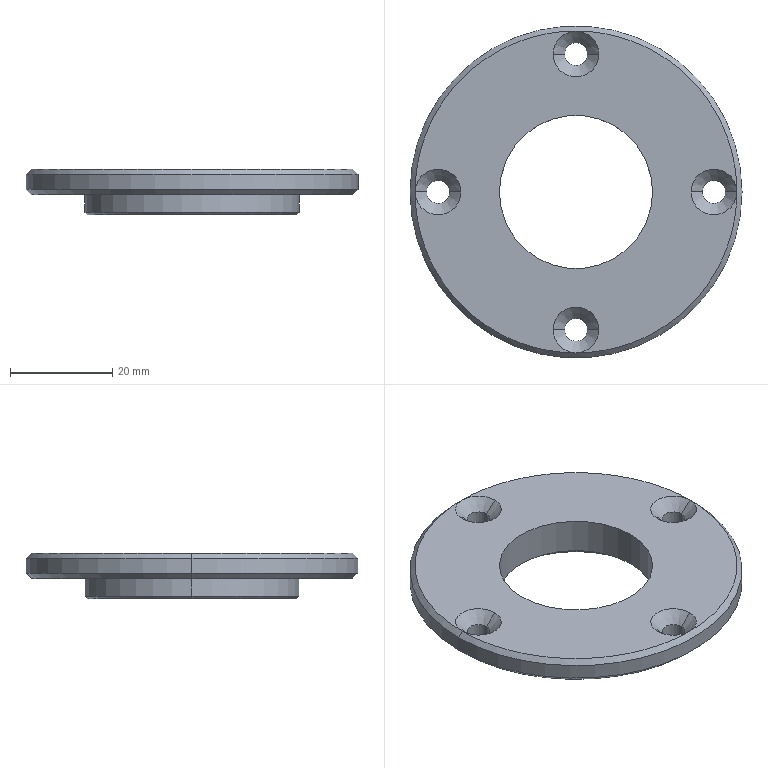Component | SolidWorks | TractionDriveWheelBearingEndCap-1 | 1 solid | 36 faces | box 65 x 65 x 9 mm | volume 14632 mm3 | cylinder 16 | cone 16 | plane 4 | commonest cylinder face diameters 4.5 x8 30 x2 34 x2 42 x2 65 x2
build123d program:
from build123d import *

# Parameters (mm, degrees)
CHAMFER1_SIZE                                        = 1
CHAMFER2_SIZE                                        = 0.5
M4_HEXAGON_SOCKET_COUNTERSUNK_HEAD_SCREW_D           = 4.5
M4_HEXAGON_SOCKET_COUNTERSUNK_HEAD_SCREW_CSINK_D     = 8.96
M4_HEXAGON_SOCKET_COUNTERSUNK_HEAD_SCREW_CSINK_ANGLE = 90
CIRPATTERN1_COUNT                                    = 4
SKETCH5_R                                            = 15
CUT_EXTRUDE1_DEPTH                                   = 47.835


with BuildPart() as part:
    # Sketch1 → Revolve1 (revolve)
    with BuildSketch(Plane(origin=(0, 0, 0), x_dir=(0, 0, -1), z_dir=(1, 0, 0)), mode=Mode.PRIVATE) as revolve1_sk:
        Polygon((0, 0), (0, 32.5), (5, 32.5), (5, 21), (9, 21), (9, 17), (7, 17), (7, 0), align=None)
    revolve(revolve1_sk.sketch.rotate(Axis((0, 0, 414.053), (0, 0, -1)), 90), axis=Axis((0, 0, 414.053), (0, 0, -1)))

    # Chamfer1
    chamfer1_edges = [part.edges().sort_by_distance(p)[0] for p in [
        (-32.5, 0, -5),
        (-32.5, 0, 0),
    ]]
    chamfer(chamfer1_edges, length=CHAMFER1_SIZE)

    # Chamfer2
    chamfer2_edges = [part.edges().sort_by_distance(p)[0] for p in [
        (-17, 0, -9),
        (-21, 0, -9),
    ]]
    chamfer(chamfer2_edges, length=CHAMFER2_SIZE)

    # M4 Hexagon Socket Countersunk Head Screw (through all)
    with Locations(Plane.XY):
        with Locations((0, 27)):
            m4_hexagon_socket_countersunk_head_screw = CounterSinkHole(M4_HEXAGON_SOCKET_COUNTERSUNK_HEAD_SCREW_D / 2, M4_HEXAGON_SOCKET_COUNTERSUNK_HEAD_SCREW_CSINK_D / 2, counter_sink_angle=M4_HEXAGON_SOCKET_COUNTERSUNK_HEAD_SCREW_CSINK_ANGLE)

    # CirPattern1: M4 Hexagon Socket Countersunk Head Screw ×4 about axis
    cirpattern1_axis = Axis((0, 0, 0), (0, 0, 1))
    for i in range(1, CIRPATTERN1_COUNT):
        add(m4_hexagon_socket_countersunk_head_screw.rotate(cirpattern1_axis, i * 360 / CIRPATTERN1_COUNT), mode=Mode.SUBTRACT)

    # Sketch5 → Cut-Extrude1 (cut, through all)
    with BuildSketch(Plane.XY):
        Circle(SKETCH5_R)
    extrude(amount=-CUT_EXTRUDE1_DEPTH, mode=Mode.SUBTRACT)


solid = part.part

# Placed as in the assembly
solid = solid.moved(Location((-299.507, -39.911, 646), (0, 0, 0)))
STEP:
#1=COLOUR_RGB('',0.7922,0.8196,0.9333);
#2=FILL_AREA_STYLE_COLOUR('',#1);
#3=FILL_AREA_STYLE('',(#2));
#4=SURFACE_STYLE_FILL_AREA(#3);
#5=SURFACE_SIDE_STYLE('',(#4));
#6=SURFACE_STYLE_USAGE(.BOTH.,#5);
#7=PRESENTATION_STYLE_ASSIGNMENT((#6));
#8=CARTESIAN_POINT('',(-12.382,-1.571,25.157));
#9=VERTEX_POINT('',#8);
#10=CARTESIAN_POINT('',(-11.201,-1.571,25.157));
#11=VERTEX_POINT('',#10);
#12=CARTESIAN_POINT('',(-11.792,-1.571,25.157));
#13=DIRECTION('',(0.,0.,1.));
#14=DIRECTION('',(1.,0.,0.));
#15=AXIS2_PLACEMENT_3D('',#12,#13,#14);
#16=CIRCLE('',#15,0.5906);
#17=EDGE_CURVE('',#9,#11,#16,.T.);
#18=ORIENTED_EDGE('',*,*,#17,.F.);
#19=CARTESIAN_POINT('',(-12.382,-1.571,25.433));
#20=VERTEX_POINT('',#19);
#21=CARTESIAN_POINT('',(-12.382,-1.571,25.079));
#22=DIRECTION('',(0.,0.,1.));
#23=VECTOR('',#22,39.37);
#24=LINE('',#21,#23);
#25=EDGE_CURVE('',#9,#20,#24,.T.);
#26=ORIENTED_EDGE('',*,*,#25,.T.);
#27=CARTESIAN_POINT('',(-11.201,-1.571,25.433));
#28=VERTEX_POINT('',#27);
#29=CARTESIAN_POINT('',(-11.792,-1.571,25.433));
#30=DIRECTION('',(0.,0.,1.));
#31=DIRECTION('',(1.,0.,0.));
#32=AXIS2_PLACEMENT_3D('',#29,#30,#31);
#33=CIRCLE('',#32,0.5906);
#34=EDGE_CURVE('',#20,#28,#33,.T.);
#35=ORIENTED_EDGE('',*,*,#34,.T.);
#36=CARTESIAN_POINT('',(-11.201,-1.571,25.079));
#37=DIRECTION('',(0.,0.,1.));
#38=VECTOR('',#37,39.37);
#39=LINE('',#36,#38);
#40=EDGE_CURVE('',#11,#28,#39,.T.);
#41=ORIENTED_EDGE('',*,*,#40,.F.);
#42=EDGE_LOOP('',(#18,#26,#35,#41));
#43=FACE_OUTER_BOUND('',#42,.T.);
#44=CARTESIAN_POINT('',(-11.792,-1.571,25.079));
#45=DIRECTION('',(0.,0.,1.));
#46=DIRECTION('',(1.,0.,0.));
#47=AXIS2_PLACEMENT_3D('',#44,#45,#46);
#48=CYLINDRICAL_SURFACE('',#47,0.5906);
#49=ADVANCED_FACE('',(#43),#48,.F.);
#50=CARTESIAN_POINT('',(-10.817,-1.571,25.345));
#51=VERTEX_POINT('',#50);
#52=CARTESIAN_POINT('',(-10.64,-1.571,25.345));
#53=VERTEX_POINT('',#52);
#54=CARTESIAN_POINT('',(-10.729,-1.571,25.345));
#55=DIRECTION('',(0.,0.,1.));
#56=DIRECTION('',(1.,0.,0.));
#57=AXIS2_PLACEMENT_3D('',#54,#55,#56);
#58=CIRCLE('',#57,0.08858);
#59=EDGE_CURVE('',#51,#53,#58,.T.);
#60=ORIENTED_EDGE('',*,*,#59,.F.);
#61=CARTESIAN_POINT('',(-10.905,-1.571,25.433));
#62=VERTEX_POINT('',#61);
#63=CARTESIAN_POINT('',(-10.905,-1.571,25.433));
#64=DIRECTION('',(-0.7071,0.,0.7071));
#65=VECTOR('',#64,39.37);
#66=LINE('',#63,#65);
#67=EDGE_CURVE('',#51,#62,#66,.T.);
#68=ORIENTED_EDGE('',*,*,#67,.T.);
#69=CARTESIAN_POINT('',(-10.552,-1.571,25.433));
#70=VERTEX_POINT('',#69);
#71=CARTESIAN_POINT('',(-10.729,-1.571,25.433));
#72=DIRECTION('',(0.,0.,1.));
#73=DIRECTION('',(1.,0.,0.));
#74=AXIS2_PLACEMENT_3D('',#71,#72,#73);
#75=CIRCLE('',#74,0.1764);
#76=EDGE_CURVE('',#62,#70,#75,.T.);
#77=ORIENTED_EDGE('',*,*,#76,.T.);
#78=CARTESIAN_POINT('',(-10.552,-1.571,25.433));
#79=DIRECTION('',(0.7071,0.,0.7071));
#80=VECTOR('',#79,39.37);
#81=LINE('',#78,#80);
#82=EDGE_CURVE('',#53,#70,#81,.T.);
#83=ORIENTED_EDGE('',*,*,#82,.F.);
#84=EDGE_LOOP('',(#60,#68,#77,#83));
#85=FACE_OUTER_BOUND('',#84,.T.);
#86=CARTESIAN_POINT('',(-10.729,-1.571,25.433));
#87=DIRECTION('',(0.,0.,1.));
#88=DIRECTION('',(1.,0.,0.));
#89=AXIS2_PLACEMENT_3D('',#86,#87,#88);
#90=CONICAL_SURFACE('',#89,0.1764,0.7854);
#91=ADVANCED_FACE('',(#85),#90,.F.);
#92=CARTESIAN_POINT('',(-10.817,-1.571,25.236));
#93=VERTEX_POINT('',#92);
#94=CARTESIAN_POINT('',(-10.64,-1.571,25.236));
#95=VERTEX_POINT('',#94);
#96=CARTESIAN_POINT('',(-10.729,-1.571,25.236));
#97=DIRECTION('',(0.,0.,1.));
#98=DIRECTION('',(1.,0.,0.));
#99=AXIS2_PLACEMENT_3D('',#96,#97,#98);
#100=CIRCLE('',#99,0.08858);
#101=EDGE_CURVE('',#93,#95,#100,.T.);
#102=ORIENTED_EDGE('',*,*,#101,.F.);
#103=CARTESIAN_POINT('',(-10.817,-1.571,25.433));
#104=DIRECTION('',(0.,0.,1.));
#105=VECTOR('',#104,39.37);
#106=LINE('',#103,#105);
#107=EDGE_CURVE('',#93,#51,#106,.T.);
#108=ORIENTED_EDGE('',*,*,#107,.T.);
#109=ORIENTED_EDGE('',*,*,#59,.T.);
#110=CARTESIAN_POINT('',(-10.64,-1.571,25.433));
#111=DIRECTION('',(0.,0.,1.));
#112=VECTOR('',#111,39.37);
#113=LINE('',#110,#112);
#114=EDGE_CURVE('',#95,#53,#113,.T.);
#115=ORIENTED_EDGE('',*,*,#114,.F.);
#116=EDGE_LOOP('',(#102,#108,#109,#115));
#117=FACE_OUTER_BOUND('',#116,.T.);
#118=CARTESIAN_POINT('',(-10.729,-1.571,25.433));
#119=DIRECTION('',(0.,0.,1.));
#120=DIRECTION('',(1.,0.,0.));
#121=AXIS2_PLACEMENT_3D('',#118,#119,#120);
#122=CYLINDRICAL_SURFACE('',#121,0.08858);
#123=ADVANCED_FACE('',(#117),#122,.F.);
#124=CARTESIAN_POINT('',(-11.88,-2.634,25.345));
#125=VERTEX_POINT('',#124);
#126=CARTESIAN_POINT('',(-11.703,-2.634,25.345));
#127=VERTEX_POINT('',#126);
#128=CARTESIAN_POINT('',(-11.792,-2.634,25.345));
#129=DIRECTION('',(0.,0.,1.));
#130=DIRECTION('',(1.,0.,0.));
#131=AXIS2_PLACEMENT_3D('',#128,#129,#130);
#132=CIRCLE('',#131,0.08858);
#133=EDGE_CURVE('',#125,#127,#132,.T.);
#134=ORIENTED_EDGE('',*,*,#133,.F.);
#135=CARTESIAN_POINT('',(-11.968,-2.634,25.433));
#136=VERTEX_POINT('',#135);
#137=CARTESIAN_POINT('',(-11.968,-2.634,25.433));
#138=DIRECTION('',(-0.7071,0.,0.7071));
#139=VECTOR('',#138,39.37);
#140=LINE('',#137,#139);
#141=EDGE_CURVE('',#125,#136,#140,.T.);
#142=ORIENTED_EDGE('',*,*,#141,.T.);
#143=CARTESIAN_POINT('',(-11.615,-2.634,25.433));
#144=VERTEX_POINT('',#143);
#145=CARTESIAN_POINT('',(-11.792,-2.634,25.433));
#146=DIRECTION('',(0.,0.,1.));
#147=DIRECTION('',(1.,0.,0.));
#148=AXIS2_PLACEMENT_3D('',#145,#146,#147);
#149=CIRCLE('',#148,0.1764);
#150=EDGE_CURVE('',#136,#144,#149,.T.);
#151=ORIENTED_EDGE('',*,*,#150,.T.);
#152=CARTESIAN_POINT('',(-11.615,-2.634,25.433));
#153=DIRECTION('',(0.7071,0.,0.7071));
#154=VECTOR('',#153,39.37);
#155=LINE('',#152,#154);
#156=EDGE_CURVE('',#127,#144,#155,.T.);
#157=ORIENTED_EDGE('',*,*,#156,.F.);
#158=EDGE_LOOP('',(#134,#142,#151,#157));
#159=FACE_OUTER_BOUND('',#158,.T.);
#160=CARTESIAN_POINT('',(-11.792,-2.634,25.433));
#161=DIRECTION('',(0.,0.,1.));
#162=DIRECTION('',(1.,0.,0.));
#163=AXIS2_PLACEMENT_3D('',#160,#161,#162);
#164=CONICAL_SURFACE('',#163,0.1764,0.7854);
#165=ADVANCED_FACE('',(#159),#164,.F.);
#166=CARTESIAN_POINT('',(-11.88,-2.634,25.236));
#167=VERTEX_POINT('',#166);
#168=CARTESIAN_POINT('',(-11.703,-2.634,25.236));
#169=VERTEX_POINT('',#168);
#170=CARTESIAN_POINT('',(-11.792,-2.634,25.236));
#171=DIRECTION('',(0.,0.,1.));
#172=DIRECTION('',(1.,0.,0.));
#173=AXIS2_PLACEMENT_3D('',#170,#171,#172);
#174=CIRCLE('',#173,0.08858);
#175=EDGE_CURVE('',#167,#169,#174,.T.);
#176=ORIENTED_EDGE('',*,*,#175,.F.);
#177=CARTESIAN_POINT('',(-11.88,-2.634,25.433));
#178=DIRECTION('',(0.,0.,1.));
#179=VECTOR('',#178,39.37);
#180=LINE('',#177,#179);
#181=EDGE_CURVE('',#167,#125,#180,.T.);
#182=ORIENTED_EDGE('',*,*,#181,.T.);
#183=ORIENTED_EDGE('',*,*,#133,.T.);
#184=CARTESIAN_POINT('',(-11.703,-2.634,25.433));
#185=DIRECTION('',(0.,0.,1.));
#186=VECTOR('',#185,39.37);
#187=LINE('',#184,#186);
#188=EDGE_CURVE('',#169,#127,#187,.T.);
#189=ORIENTED_EDGE('',*,*,#188,.F.);
#190=EDGE_LOOP('',(#176,#182,#183,#189));
#191=FACE_OUTER_BOUND('',#190,.T.);
#192=CARTESIAN_POINT('',(-11.792,-2.634,25.433));
#193=DIRECTION('',(0.,0.,1.));
#194=DIRECTION('',(1.,0.,0.));
#195=AXIS2_PLACEMENT_3D('',#192,#193,#194);
#196=CYLINDRICAL_SURFACE('',#195,0.08858);
#197=ADVANCED_FACE('',(#191),#196,.F.);
#198=CARTESIAN_POINT('',(-12.943,-1.571,25.345));
#199=VERTEX_POINT('',#198);
#200=CARTESIAN_POINT('',(-12.766,-1.571,25.345));
#201=VERTEX_POINT('',#200);
#202=CARTESIAN_POINT('',(-12.855,-1.571,25.345));
#203=DIRECTION('',(0.,0.,1.));
#204=DIRECTION('',(1.,0.,0.));
#205=AXIS2_PLACEMENT_3D('',#202,#203,#204);
#206=CIRCLE('',#205,0.08858);
#207=EDGE_CURVE('',#199,#201,#206,.T.);
#208=ORIENTED_EDGE('',*,*,#207,.F.);
#209=CARTESIAN_POINT('',(-13.031,-1.571,25.433));
#210=VERTEX_POINT('',#209);
#211=CARTESIAN_POINT('',(-13.031,-1.571,25.433));
#212=DIRECTION('',(-0.7071,0.,0.7071));
#213=VECTOR('',#212,39.37);
#214=LINE('',#211,#213);
#215=EDGE_CURVE('',#199,#210,#214,.T.);
#216=ORIENTED_EDGE('',*,*,#215,.T.);
#217=CARTESIAN_POINT('',(-12.678,-1.571,25.433));
#218=VERTEX_POINT('',#217);
#219=CARTESIAN_POINT('',(-12.855,-1.571,25.433));
#220=DIRECTION('',(0.,0.,1.));
#221=DIRECTION('',(1.,0.,0.));
#222=AXIS2_PLACEMENT_3D('',#219,#220,#221);
#223=CIRCLE('',#222,0.1764);
#224=EDGE_CURVE('',#210,#218,#223,.T.);
#225=ORIENTED_EDGE('',*,*,#224,.T.);
#226=CARTESIAN_POINT('',(-12.678,-1.571,25.433));
#227=DIRECTION('',(0.7071,0.,0.7071));
#228=VECTOR('',#227,39.37);
#229=LINE('',#226,#228);
#230=EDGE_CURVE('',#201,#218,#229,.T.);
#231=ORIENTED_EDGE('',*,*,#230,.F.);
#232=EDGE_LOOP('',(#208,#216,#225,#231));
#233=FACE_OUTER_BOUND('',#232,.T.);
#234=CARTESIAN_POINT('',(-12.855,-1.571,25.433));
#235=DIRECTION('',(0.,0.,1.));
#236=DIRECTION('',(1.,0.,0.));
#237=AXIS2_PLACEMENT_3D('',#234,#235,#236);
#238=CONICAL_SURFACE('',#237,0.1764,0.7854);
#239=ADVANCED_FACE('',(#233),#238,.F.);
#240=CARTESIAN_POINT('',(-12.943,-1.571,25.236));
#241=VERTEX_POINT('',#240);
#242=CARTESIAN_POINT('',(-12.766,-1.571,25.236));
#243=VERTEX_POINT('',#242);
#244=CARTESIAN_POINT('',(-12.855,-1.571,25.236));
#245=DIRECTION('',(0.,0.,1.));
#246=DIRECTION('',(1.,0.,0.));
#247=AXIS2_PLACEMENT_3D('',#244,#245,#246);
#248=CIRCLE('',#247,0.08858);
#249=EDGE_CURVE('',#241,#243,#248,.T.);
#250=ORIENTED_EDGE('',*,*,#249,.F.);
#251=CARTESIAN_POINT('',(-12.943,-1.571,25.433));
#252=DIRECTION('',(0.,0.,1.));
#253=VECTOR('',#252,39.37);
#254=LINE('',#251,#253);
#255=EDGE_CURVE('',#241,#199,#254,.T.);
#256=ORIENTED_EDGE('',*,*,#255,.T.);
#257=ORIENTED_EDGE('',*,*,#207,.T.);
#258=CARTESIAN_POINT('',(-12.766,-1.571,25.433));
#259=DIRECTION('',(0.,0.,1.));
#260=VECTOR('',#259,39.37);
#261=LINE('',#258,#260);
#262=EDGE_CURVE('',#243,#201,#261,.T.);
#263=ORIENTED_EDGE('',*,*,#262,.F.);
#264=EDGE_LOOP('',(#250,#256,#257,#263));
#265=FACE_OUTER_BOUND('',#264,.T.);
#266=CARTESIAN_POINT('',(-12.855,-1.571,25.433));
#267=DIRECTION('',(0.,0.,1.));
#268=DIRECTION('',(1.,0.,0.));
#269=AXIS2_PLACEMENT_3D('',#266,#267,#268);
#270=CYLINDRICAL_SURFACE('',#269,0.08858);
#271=ADVANCED_FACE('',(#265),#270,.F.);
#272=CARTESIAN_POINT('',(-11.88,-0.5083,25.345));
#273=VERTEX_POINT('',#272);
#274=CARTESIAN_POINT('',(-11.703,-0.5083,25.345));
#275=VERTEX_POINT('',#274);
#276=CARTESIAN_POINT('',(-11.792,-0.5083,25.345));
#277=DIRECTION('',(0.,0.,1.));
#278=DIRECTION('',(1.,0.,0.));
#279=AXIS2_PLACEMENT_3D('',#276,#277,#278);
#280=CIRCLE('',#279,0.08858);
#281=EDGE_CURVE('',#273,#275,#280,.T.);
#282=ORIENTED_EDGE('',*,*,#281,.F.);
#283=CARTESIAN_POINT('',(-11.968,-0.5083,25.433));
#284=VERTEX_POINT('',#283);
#285=CARTESIAN_POINT('',(-11.968,-0.5083,25.433));
#286=DIRECTION('',(-0.7071,0.,0.7071));
#287=VECTOR('',#286,39.37);
#288=LINE('',#285,#287);
#289=EDGE_CURVE('',#273,#284,#288,.T.);
#290=ORIENTED_EDGE('',*,*,#289,.T.);
#291=CARTESIAN_POINT('',(-11.615,-0.5083,25.433));
#292=VERTEX_POINT('',#291);
#293=CARTESIAN_POINT('',(-11.792,-0.5083,25.433));
#294=DIRECTION('',(0.,0.,1.));
#295=DIRECTION('',(1.,0.,0.));
#296=AXIS2_PLACEMENT_3D('',#293,#294,#295);
#297=CIRCLE('',#296,0.1764);
#298=EDGE_CURVE('',#284,#292,#297,.T.);
#299=ORIENTED_EDGE('',*,*,#298,.T.);
#300=CARTESIAN_POINT('',(-11.615,-0.5083,25.433));
#301=DIRECTION('',(0.7071,0.,0.7071));
#302=VECTOR('',#301,39.37);
#303=LINE('',#300,#302);
#304=EDGE_CURVE('',#275,#292,#303,.T.);
#305=ORIENTED_EDGE('',*,*,#304,.F.);
#306=EDGE_LOOP('',(#282,#290,#299,#305));
#307=FACE_OUTER_BOUND('',#306,.T.);
#308=CARTESIAN_POINT('',(-11.792,-0.5083,25.433));
#309=DIRECTION('',(0.,0.,1.));
#310=DIRECTION('',(1.,0.,0.));
#311=AXIS2_PLACEMENT_3D('',#308,#309,#310);
#312=CONICAL_SURFACE('',#311,0.1764,0.7854);
#313=ADVANCED_FACE('',(#307),#312,.F.);
#314=CARTESIAN_POINT('',(-11.88,-0.5083,25.236));
#315=VERTEX_POINT('',#314);
#316=CARTESIAN_POINT('',(-11.703,-0.5083,25.236));
#317=VERTEX_POINT('',#316);
#318=CARTESIAN_POINT('',(-11.792,-0.5083,25.236));
#319=DIRECTION('',(0.,0.,1.));
#320=DIRECTION('',(1.,0.,0.));
#321=AXIS2_PLACEMENT_3D('',#318,#319,#320);
#322=CIRCLE('',#321,0.08858);
#323=EDGE_CURVE('',#315,#317,#322,.T.);
#324=ORIENTED_EDGE('',*,*,#323,.F.);
#325=CARTESIAN_POINT('',(-11.88,-0.5083,25.433));
#326=DIRECTION('',(0.,0.,1.));
#327=VECTOR('',#326,39.37);
#328=LINE('',#325,#327);
#329=EDGE_CURVE('',#315,#273,#328,.T.);
#330=ORIENTED_EDGE('',*,*,#329,.T.);
#331=ORIENTED_EDGE('',*,*,#281,.T.);
#332=CARTESIAN_POINT('',(-11.703,-0.5083,25.433));
#333=DIRECTION('',(0.,0.,1.));
#334=VECTOR('',#333,39.37);
#335=LINE('',#332,#334);
#336=EDGE_CURVE('',#317,#275,#335,.T.);
#337=ORIENTED_EDGE('',*,*,#336,.F.);
#338=EDGE_LOOP('',(#324,#330,#331,#337));
#339=FACE_OUTER_BOUND('',#338,.T.);
#340=CARTESIAN_POINT('',(-11.792,-0.5083,25.433));
#341=DIRECTION('',(0.,0.,1.));
#342=DIRECTION('',(1.,0.,0.));
#343=AXIS2_PLACEMENT_3D('',#340,#341,#342);
#344=CYLINDRICAL_SURFACE('',#343,0.08858);
#345=ADVANCED_FACE('',(#339),#344,.F.);
#346=CARTESIAN_POINT('',(-11.122,-1.571,25.098));
#347=VERTEX_POINT('',#346);
#348=CARTESIAN_POINT('',(-12.461,-1.571,25.098));
#349=VERTEX_POINT('',#348);
#350=CARTESIAN_POINT('',(-11.792,-1.571,25.098));
#351=DIRECTION('',(0.,0.,-1.));
#352=DIRECTION('',(1.,0.,0.));
#353=AXIS2_PLACEMENT_3D('',#350,#351,#352);
#354=CIRCLE('',#353,0.6693);
#355=EDGE_CURVE('',#347,#349,#354,.T.);
#356=ORIENTED_EDGE('',*,*,#355,.F.);
#357=CARTESIAN_POINT('',(-11.103,-1.571,25.079));
#358=VERTEX_POINT('',#357);
#359=CARTESIAN_POINT('',(-11.103,-1.571,25.079));
#360=DIRECTION('',(0.7071,0.,-0.7071));
#361=VECTOR('',#360,39.37);
#362=LINE('',#359,#361);
#363=EDGE_CURVE('',#347,#358,#362,.T.);
#364=ORIENTED_EDGE('',*,*,#363,.T.);
#365=CARTESIAN_POINT('',(-12.481,-1.571,25.079));
#366=VERTEX_POINT('',#365);
#367=CARTESIAN_POINT('',(-11.792,-1.571,25.079));
#368=DIRECTION('',(0.,0.,1.));
#369=DIRECTION('',(1.,0.,0.));
#370=AXIS2_PLACEMENT_3D('',#367,#368,#369);
#371=CIRCLE('',#370,0.689);
#372=EDGE_CURVE('',#366,#358,#371,.T.);
#373=ORIENTED_EDGE('',*,*,#372,.F.);
#374=CARTESIAN_POINT('',(-12.481,-1.571,25.079));
#375=DIRECTION('',(-0.7071,0.,-0.7071));
#376=VECTOR('',#375,39.37);
#377=LINE('',#374,#376);
#378=EDGE_CURVE('',#349,#366,#377,.T.);
#379=ORIENTED_EDGE('',*,*,#378,.F.);
#380=EDGE_LOOP('',(#356,#364,#373,#379));
#381=FACE_OUTER_BOUND('',#380,.T.);
#382=CARTESIAN_POINT('',(-11.792,-1.571,25.079));
#383=DIRECTION('',(0.,0.,-1.));
#384=DIRECTION('',(-1.,0.,0.));
#385=AXIS2_PLACEMENT_3D('',#382,#383,#384);
#386=CONICAL_SURFACE('',#385,0.689,0.7854);
#387=ADVANCED_FACE('',(#381),#386,.F.);
#388=CARTESIAN_POINT('',(-12.599,-1.571,25.079));
#389=VERTEX_POINT('',#388);
#390=CARTESIAN_POINT('',(-10.985,-1.571,25.079));
#391=VERTEX_POINT('',#390);
#392=CARTESIAN_POINT('',(-11.792,-1.571,25.079));
#393=DIRECTION('',(0.,0.,-1.));
#394=DIRECTION('',(1.,0.,0.));
#395=AXIS2_PLACEMENT_3D('',#392,#393,#394);
#396=CIRCLE('',#395,0.8071);
#397=EDGE_CURVE('',#389,#391,#396,.T.);
#398=ORIENTED_EDGE('',*,*,#397,.F.);
#399=CARTESIAN_POINT('',(-12.618,-1.571,25.098));
#400=VERTEX_POINT('',#399);
#401=CARTESIAN_POINT('',(-12.618,-1.571,25.098));
#402=DIRECTION('',(-0.7071,0.,0.7071));
#403=VECTOR('',#402,39.37);
#404=LINE('',#401,#403);
#405=EDGE_CURVE('',#389,#400,#404,.T.);
#406=ORIENTED_EDGE('',*,*,#405,.T.);
#407=CARTESIAN_POINT('',(-10.965,-1.571,25.098));
#408=VERTEX_POINT('',#407);
#409=CARTESIAN_POINT('',(-11.792,-1.571,25.098));
#410=DIRECTION('',(0.,0.,1.));
#411=DIRECTION('',(1.,0.,0.));
#412=AXIS2_PLACEMENT_3D('',#409,#410,#411);
#413=CIRCLE('',#412,0.8268);
#414=EDGE_CURVE('',#408,#400,#413,.T.);
#415=ORIENTED_EDGE('',*,*,#414,.F.);
#416=CARTESIAN_POINT('',(-10.965,-1.571,25.098));
#417=DIRECTION('',(0.7071,0.,0.7071));
#418=VECTOR('',#417,39.37);
#419=LINE('',#416,#418);
#420=EDGE_CURVE('',#391,#408,#419,.T.);
#421=ORIENTED_EDGE('',*,*,#420,.F.);
#422=EDGE_LOOP('',(#398,#406,#415,#421));
#423=FACE_OUTER_BOUND('',#422,.T.);
#424=CARTESIAN_POINT('',(-11.792,-1.571,25.098));
#425=DIRECTION('',(0.,0.,1.));
#426=DIRECTION('',(1.,0.,0.));
#427=AXIS2_PLACEMENT_3D('',#424,#425,#426);
#428=CONICAL_SURFACE('',#427,0.8268,0.7854);
#429=ADVANCED_FACE('',(#423),#428,.T.);
#430=CARTESIAN_POINT('',(-13.032,-1.571,25.236));
#431=VERTEX_POINT('',#430);
#432=CARTESIAN_POINT('',(-10.551,-1.571,25.236));
#433=VERTEX_POINT('',#432);
#434=CARTESIAN_POINT('',(-11.792,-1.571,25.236));
#435=DIRECTION('',(0.,0.,-1.));
#436=DIRECTION('',(1.,0.,0.));
#437=AXIS2_PLACEMENT_3D('',#434,#435,#436);
#438=CIRCLE('',#437,1.24);
#439=EDGE_CURVE('',#431,#433,#438,.T.);
#440=ORIENTED_EDGE('',*,*,#439,.F.);
#441=CARTESIAN_POINT('',(-13.071,-1.571,25.276));
#442=VERTEX_POINT('',#441);
#443=CARTESIAN_POINT('',(-13.071,-1.571,25.276));
#444=DIRECTION('',(-0.7071,0.,0.7071));
#445=VECTOR('',#444,39.37);
#446=LINE('',#443,#445);
#447=EDGE_CURVE('',#431,#442,#446,.T.);
#448=ORIENTED_EDGE('',*,*,#447,.T.);
#449=CARTESIAN_POINT('',(-10.512,-1.571,25.276));
#450=VERTEX_POINT('',#449);
#451=CARTESIAN_POINT('',(-11.792,-1.571,25.276));
#452=DIRECTION('',(0.,0.,1.));
#453=DIRECTION('',(1.,0.,0.));
#454=AXIS2_PLACEMENT_3D('',#451,#452,#453);
#455=CIRCLE('',#454,1.28);
#456=EDGE_CURVE('',#450,#442,#455,.T.);
#457=ORIENTED_EDGE('',*,*,#456,.F.);
#458=CARTESIAN_POINT('',(-10.512,-1.571,25.276));
#459=DIRECTION('',(0.7071,0.,0.7071));
#460=VECTOR('',#459,39.37);
#461=LINE('',#458,#460);
#462=EDGE_CURVE('',#433,#450,#461,.T.);
#463=ORIENTED_EDGE('',*,*,#462,.F.);
#464=EDGE_LOOP('',(#440,#448,#457,#463));
#465=FACE_OUTER_BOUND('',#464,.T.);
#466=CARTESIAN_POINT('',(-11.792,-1.571,25.276));
#467=DIRECTION('',(0.,0.,1.));
#468=DIRECTION('',(1.,0.,0.));
#469=AXIS2_PLACEMENT_3D('',#466,#467,#468);
#470=CONICAL_SURFACE('',#469,1.28,0.7854);
#471=ADVANCED_FACE('',(#465),#470,.T.);
#472=CARTESIAN_POINT('',(-10.551,-1.571,25.433));
#473=VERTEX_POINT('',#472);
#474=CARTESIAN_POINT('',(-13.032,-1.571,25.433));
#475=VERTEX_POINT('',#474);
#476=CARTESIAN_POINT('',(-11.792,-1.571,25.433));
#477=DIRECTION('',(0.,0.,1.));
#478=DIRECTION('',(-1.,0.,0.));
#479=AXIS2_PLACEMENT_3D('',#476,#477,#478);
#480=CIRCLE('',#479,1.24);
#481=EDGE_CURVE('',#473,#475,#480,.T.);
#482=ORIENTED_EDGE('',*,*,#481,.F.);
#483=CARTESIAN_POINT('',(-10.512,-1.571,25.394));
#484=VERTEX_POINT('',#483);
#485=CARTESIAN_POINT('',(-10.551,-1.571,25.433));
#486=DIRECTION('',(0.7071,0.,-0.7071));
#487=VECTOR('',#486,39.37);
#488=LINE('',#485,#487);
#489=EDGE_CURVE('',#473,#484,#488,.T.);
#490=ORIENTED_EDGE('',*,*,#489,.T.);
#491=CARTESIAN_POINT('',(-13.071,-1.571,25.394));
#492=VERTEX_POINT('',#491);
#493=CARTESIAN_POINT('',(-11.792,-1.571,25.394));
#494=DIRECTION('',(0.,0.,-1.));
#495=DIRECTION('',(-1.,0.,0.));
#496=AXIS2_PLACEMENT_3D('',#493,#494,#495);
#497=CIRCLE('',#496,1.28);
#498=EDGE_CURVE('',#492,#484,#497,.T.);
#499=ORIENTED_EDGE('',*,*,#498,.F.);
#500=CARTESIAN_POINT('',(-13.032,-1.571,25.433));
#501=DIRECTION('',(-0.7071,0.,-0.7071));
#502=VECTOR('',#501,39.37);
#503=LINE('',#500,#502);
#504=EDGE_CURVE('',#475,#492,#503,.T.);
#505=ORIENTED_EDGE('',*,*,#504,.F.);
#506=EDGE_LOOP('',(#482,#490,#499,#505));
#507=FACE_OUTER_BOUND('',#506,.T.);
#508=CARTESIAN_POINT('',(-11.792,-1.571,25.433));
#509=DIRECTION('',(0.,0.,-1.));
#510=DIRECTION('',(-1.,0.,0.));
#511=AXIS2_PLACEMENT_3D('',#508,#509,#510);
#512=CONICAL_SURFACE('',#511,1.24,0.7854);
#513=ADVANCED_FACE('',(#507),#512,.T.);
#514=ORIENTED_EDGE('',*,*,#355,.T.);
#515=CARTESIAN_POINT('',(-12.461,-1.571,25.157));
#516=VERTEX_POINT('',#515);
#517=CARTESIAN_POINT('',(-12.461,-1.571,41.734));
#518=DIRECTION('',(0.,0.,1.));
#519=VECTOR('',#518,39.37);
#520=LINE('',#517,#519);
#521=EDGE_CURVE('',#349,#516,#520,.T.);
#522=ORIENTED_EDGE('',*,*,#521,.T.);
#523=CARTESIAN_POINT('',(-11.122,-1.571,25.157));
#524=VERTEX_POINT('',#523);
#525=CARTESIAN_POINT('',(-11.792,-1.571,25.157));
#526=DIRECTION('',(0.,0.,1.));
#527=DIRECTION('',(1.,0.,0.));
#528=AXIS2_PLACEMENT_3D('',#525,#526,#527);
#529=CIRCLE('',#528,0.6693);
#530=EDGE_CURVE('',#516,#524,#529,.T.);
#531=ORIENTED_EDGE('',*,*,#530,.T.);
#532=CARTESIAN_POINT('',(-11.122,-1.571,41.734));
#533=DIRECTION('',(0.,0.,1.));
#534=VECTOR('',#533,39.37);
#535=LINE('',#532,#534);
#536=EDGE_CURVE('',#347,#524,#535,.T.);
#537=ORIENTED_EDGE('',*,*,#536,.F.);
#538=EDGE_LOOP('',(#514,#522,#531,#537));
#539=FACE_OUTER_BOUND('',#538,.T.);
#540=CARTESIAN_POINT('',(-11.792,-1.571,41.734));
#541=DIRECTION('',(0.,0.,1.));
#542=DIRECTION('',(1.,0.,0.));
#543=AXIS2_PLACEMENT_3D('',#540,#541,#542);
#544=CYLINDRICAL_SURFACE('',#543,0.6693);
#545=ADVANCED_FACE('',(#539),#544,.F.);
#546=ORIENTED_EDGE('',*,*,#414,.T.);
#547=CARTESIAN_POINT('',(-12.618,-1.571,25.236));
#548=VERTEX_POINT('',#547);
#549=CARTESIAN_POINT('',(-12.618,-1.571,41.734));
#550=DIRECTION('',(0.,0.,1.));
#551=VECTOR('',#550,39.37);
#552=LINE('',#549,#551);
#553=EDGE_CURVE('',#400,#548,#552,.T.);
#554=ORIENTED_EDGE('',*,*,#553,.T.);
#555=CARTESIAN_POINT('',(-10.965,-1.571,25.236));
#556=VERTEX_POINT('',#555);
#557=CARTESIAN_POINT('',(-11.792,-1.571,25.236));
#558=DIRECTION('',(0.,0.,1.));
#559=DIRECTION('',(1.,0.,0.));
#560=AXIS2_PLACEMENT_3D('',#557,#558,#559);
#561=CIRCLE('',#560,0.8268);
#562=EDGE_CURVE('',#556,#548,#561,.T.);
#563=ORIENTED_EDGE('',*,*,#562,.F.);
#564=CARTESIAN_POINT('',(-10.965,-1.571,41.734));
#565=DIRECTION('',(0.,0.,1.));
#566=VECTOR('',#565,39.37);
#567=LINE('',#564,#566);
#568=EDGE_CURVE('',#408,#556,#567,.T.);
#569=ORIENTED_EDGE('',*,*,#568,.F.);
#570=EDGE_LOOP('',(#546,#554,#563,#569));
#571=FACE_OUTER_BOUND('',#570,.T.);
#572=CARTESIAN_POINT('',(-11.792,-1.571,41.734));
#573=DIRECTION('',(0.,0.,1.));
#574=DIRECTION('',(1.,0.,0.));
#575=AXIS2_PLACEMENT_3D('',#572,#573,#574);
#576=CYLINDRICAL_SURFACE('',#575,0.8268);
#577=ADVANCED_FACE('',(#571),#576,.T.);
#578=ORIENTED_EDGE('',*,*,#456,.T.);
#579=CARTESIAN_POINT('',(-13.071,-1.571,41.734));
#580=DIRECTION('',(0.,0.,1.));
#581=VECTOR('',#580,39.37);
#582=LINE('',#579,#581);
#583=EDGE_CURVE('',#442,#492,#582,.T.);
#584=ORIENTED_EDGE('',*,*,#583,.T.);
#585=ORIENTED_EDGE('',*,*,#498,.T.);
#586=CARTESIAN_POINT('',(-10.512,-1.571,41.734));
#587=DIRECTION('',(0.,0.,1.));
#588=VECTOR('',#587,39.37);
#589=LINE('',#586,#588);
#590=EDGE_CURVE('',#450,#484,#589,.T.);
#591=ORIENTED_EDGE('',*,*,#590,.F.);
#592=EDGE_LOOP('',(#578,#584,#585,#591));
#593=FACE_OUTER_BOUND('',#592,.T.);
#594=CARTESIAN_POINT('',(-11.792,-1.571,41.734));
#595=DIRECTION('',(0.,0.,1.));
#596=DIRECTION('',(1.,0.,0.));
#597=AXIS2_PLACEMENT_3D('',#594,#595,#596);
#598=CYLINDRICAL_SURFACE('',#597,1.28);
#599=ADVANCED_FACE('',(#593),#598,.T.);
#600=CARTESIAN_POINT('',(-11.792,-1.571,25.433));
#601=DIRECTION('',(0.,0.,1.));
#602=DIRECTION('',(1.,0.,0.));
#603=AXIS2_PLACEMENT_3D('',#600,#601,#602);
#604=CIRCLE('',#603,0.5906);
#605=EDGE_CURVE('',#28,#20,#604,.T.);
#606=ORIENTED_EDGE('',*,*,#605,.F.);
#607=ORIENTED_EDGE('',*,*,#34,.F.);
#608=EDGE_LOOP('',(#606,#607));
#609=FACE_BOUND('',#608,.T.);
#610=CARTESIAN_POINT('',(-10.729,-1.571,25.433));
#611=DIRECTION('',(0.,0.,1.));
#612=DIRECTION('',(1.,0.,0.));
#613=AXIS2_PLACEMENT_3D('',#610,#611,#612);
#614=CIRCLE('',#613,0.1764);
#615=EDGE_CURVE('',#70,#62,#614,.T.);
#616=ORIENTED_EDGE('',*,*,#615,.F.);
#617=ORIENTED_EDGE('',*,*,#76,.F.);
#618=EDGE_LOOP('',(#616,#617));
#619=FACE_BOUND('',#618,.T.);
#620=CARTESIAN_POINT('',(-11.792,-2.634,25.433));
#621=DIRECTION('',(0.,0.,1.));
#622=DIRECTION('',(1.,0.,0.));
#623=AXIS2_PLACEMENT_3D('',#620,#621,#622);
#624=CIRCLE('',#623,0.1764);
#625=EDGE_CURVE('',#144,#136,#624,.T.);
#626=ORIENTED_EDGE('',*,*,#625,.F.);
#627=ORIENTED_EDGE('',*,*,#150,.F.);
#628=EDGE_LOOP('',(#626,#627));
#629=FACE_BOUND('',#628,.T.);
#630=CARTESIAN_POINT('',(-12.855,-1.571,25.433));
#631=DIRECTION('',(0.,0.,1.));
#632=DIRECTION('',(1.,0.,0.));
#633=AXIS2_PLACEMENT_3D('',#630,#631,#632);
#634=CIRCLE('',#633,0.1764);
#635=EDGE_CURVE('',#218,#210,#634,.T.);
#636=ORIENTED_EDGE('',*,*,#635,.F.);
#637=ORIENTED_EDGE('',*,*,#224,.F.);
#638=EDGE_LOOP('',(#636,#637));
#639=FACE_BOUND('',#638,.T.);
#640=CARTESIAN_POINT('',(-11.792,-0.5083,25.433));
#641=DIRECTION('',(0.,0.,1.));
#642=DIRECTION('',(1.,0.,0.));
#643=AXIS2_PLACEMENT_3D('',#640,#641,#642);
#644=CIRCLE('',#643,0.1764);
#645=EDGE_CURVE('',#292,#284,#644,.T.);
#646=ORIENTED_EDGE('',*,*,#645,.F.);
#647=ORIENTED_EDGE('',*,*,#298,.F.);
#648=EDGE_LOOP('',(#646,#647));
#649=FACE_BOUND('',#648,.T.);
#650=CARTESIAN_POINT('',(-11.792,-1.571,25.433));
#651=DIRECTION('',(0.,0.,1.));
#652=DIRECTION('',(-1.,0.,0.));
#653=AXIS2_PLACEMENT_3D('',#650,#651,#652);
#654=CIRCLE('',#653,1.24);
#655=EDGE_CURVE('',#475,#473,#654,.T.);
#656=ORIENTED_EDGE('',*,*,#655,.T.);
#657=ORIENTED_EDGE('',*,*,#481,.T.);
#658=EDGE_LOOP('',(#656,#657));
#659=FACE_OUTER_BOUND('',#658,.T.);
#660=CARTESIAN_POINT('',(-11.792,-1.571,25.433));
#661=DIRECTION('',(0.,0.,-1.));
#662=DIRECTION('',(-1.,0.,0.));
#663=AXIS2_PLACEMENT_3D('',#660,#661,#662);
#664=PLANE('',#663);
#665=ADVANCED_FACE('',(#609,#619,#629,#639,#649,#659),#664,.F.);
#666=ORIENTED_EDGE('',*,*,#583,.F.);
#667=CARTESIAN_POINT('',(-11.792,-1.571,25.276));
#668=DIRECTION('',(0.,0.,1.));
#669=DIRECTION('',(1.,0.,0.));
#670=AXIS2_PLACEMENT_3D('',#667,#668,#669);
#671=CIRCLE('',#670,1.28);
#672=EDGE_CURVE('',#442,#450,#671,.T.);
#673=ORIENTED_EDGE('',*,*,#672,.T.);
#674=ORIENTED_EDGE('',*,*,#590,.T.);
#675=CARTESIAN_POINT('',(-11.792,-1.571,25.394));
#676=DIRECTION('',(0.,0.,-1.));
#677=DIRECTION('',(-1.,0.,0.));
#678=AXIS2_PLACEMENT_3D('',#675,#676,#677);
#679=CIRCLE('',#678,1.28);
#680=EDGE_CURVE('',#484,#492,#679,.T.);
#681=ORIENTED_EDGE('',*,*,#680,.T.);
#682=EDGE_LOOP('',(#666,#673,#674,#681));
#683=FACE_OUTER_BOUND('',#682,.T.);
#684=CARTESIAN_POINT('',(-11.792,-1.571,41.734));
#685=DIRECTION('',(0.,0.,1.));
#686=DIRECTION('',(1.,0.,0.));
#687=AXIS2_PLACEMENT_3D('',#684,#685,#686);
#688=CYLINDRICAL_SURFACE('',#687,1.28);
#689=ADVANCED_FACE('',(#683),#688,.T.);
#690=CARTESIAN_POINT('',(-10.729,-1.571,25.236));
#691=DIRECTION('',(0.,0.,1.));
#692=DIRECTION('',(1.,0.,0.));
#693=AXIS2_PLACEMENT_3D('',#690,#691,#692);
#694=CIRCLE('',#693,0.08858);
#695=EDGE_CURVE('',#95,#93,#694,.T.);
#696=ORIENTED_EDGE('',*,*,#695,.T.);
#697=ORIENTED_EDGE('',*,*,#101,.T.);
#698=EDGE_LOOP('',(#696,#697));
#699=FACE_BOUND('',#698,.T.);
#700=CARTESIAN_POINT('',(-11.792,-2.634,25.236));
#701=DIRECTION('',(0.,0.,1.));
#702=DIRECTION('',(1.,0.,0.));
#703=AXIS2_PLACEMENT_3D('',#700,#701,#702);
#704=CIRCLE('',#703,0.08858);
#705=EDGE_CURVE('',#169,#167,#704,.T.);
#706=ORIENTED_EDGE('',*,*,#705,.T.);
#707=ORIENTED_EDGE('',*,*,#175,.T.);
#708=EDGE_LOOP('',(#706,#707));
#709=FACE_BOUND('',#708,.T.);
#710=CARTESIAN_POINT('',(-12.855,-1.571,25.236));
#711=DIRECTION('',(0.,0.,1.));
#712=DIRECTION('',(1.,0.,0.));
#713=AXIS2_PLACEMENT_3D('',#710,#711,#712);
#714=CIRCLE('',#713,0.08858);
#715=EDGE_CURVE('',#243,#241,#714,.T.);
#716=ORIENTED_EDGE('',*,*,#715,.T.);
#717=ORIENTED_EDGE('',*,*,#249,.T.);
#718=EDGE_LOOP('',(#716,#717));
#719=FACE_BOUND('',#718,.T.);
#720=CARTESIAN_POINT('',(-11.792,-0.5083,25.236));
#721=DIRECTION('',(0.,0.,1.));
#722=DIRECTION('',(1.,0.,0.));
#723=AXIS2_PLACEMENT_3D('',#720,#721,#722);
#724=CIRCLE('',#723,0.08858);
#725=EDGE_CURVE('',#317,#315,#724,.T.);
#726=ORIENTED_EDGE('',*,*,#725,.T.);
#727=ORIENTED_EDGE('',*,*,#323,.T.);
#728=EDGE_LOOP('',(#726,#727));
#729=FACE_BOUND('',#728,.T.);
#730=CARTESIAN_POINT('',(-11.792,-1.571,25.236));
#731=DIRECTION('',(0.,0.,-1.));
#732=DIRECTION('',(1.,0.,0.));
#733=AXIS2_PLACEMENT_3D('',#730,#731,#732);
#734=CIRCLE('',#733,1.24);
#735=EDGE_CURVE('',#433,#431,#734,.T.);
#736=ORIENTED_EDGE('',*,*,#735,.T.);
#737=ORIENTED_EDGE('',*,*,#439,.T.);
#738=EDGE_LOOP('',(#736,#737));
#739=FACE_OUTER_BOUND('',#738,.T.);
#740=ORIENTED_EDGE('',*,*,#562,.T.);
#741=CARTESIAN_POINT('',(-11.792,-1.571,25.236));
#742=DIRECTION('',(0.,0.,1.));
#743=DIRECTION('',(1.,0.,0.));
#744=AXIS2_PLACEMENT_3D('',#741,#742,#743);
#745=CIRCLE('',#744,0.8268);
#746=EDGE_CURVE('',#548,#556,#745,.T.);
#747=ORIENTED_EDGE('',*,*,#746,.T.);
#748=EDGE_LOOP('',(#740,#747));
#749=FACE_BOUND('',#748,.T.);
#750=CARTESIAN_POINT('',(-11.792,-0.2918,25.236));
#751=DIRECTION('',(0.,0.,1.));
#752=DIRECTION('',(1.,0.,0.));
#753=AXIS2_PLACEMENT_3D('',#750,#751,#752);
#754=PLANE('',#753);
#755=ADVANCED_FACE('',(#699,#709,#719,#729,#739,#749),#754,.F.);
#756=ORIENTED_EDGE('',*,*,#553,.F.);
#757=CARTESIAN_POINT('',(-11.792,-1.571,25.098));
#758=DIRECTION('',(0.,0.,1.));
#759=DIRECTION('',(1.,0.,0.));
#760=AXIS2_PLACEMENT_3D('',#757,#758,#759);
#761=CIRCLE('',#760,0.8268);
#762=EDGE_CURVE('',#400,#408,#761,.T.);
#763=ORIENTED_EDGE('',*,*,#762,.T.);
#764=ORIENTED_EDGE('',*,*,#568,.T.);
#765=ORIENTED_EDGE('',*,*,#746,.F.);
#766=EDGE_LOOP('',(#756,#763,#764,#765));
#767=FACE_OUTER_BOUND('',#766,.T.);
#768=CARTESIAN_POINT('',(-11.792,-1.571,41.734));
#769=DIRECTION('',(0.,0.,1.));
#770=DIRECTION('',(1.,0.,0.));
#771=AXIS2_PLACEMENT_3D('',#768,#769,#770);
#772=CYLINDRICAL_SURFACE('',#771,0.8268);
#773=ADVANCED_FACE('',(#767),#772,.T.);
#774=CARTESIAN_POINT('',(-11.792,-1.571,25.079));
#775=DIRECTION('',(0.,0.,-1.));
#776=DIRECTION('',(1.,0.,0.));
#777=AXIS2_PLACEMENT_3D('',#774,#775,#776);
#778=CIRCLE('',#777,0.8071);
#779=EDGE_CURVE('',#391,#389,#778,.T.);
#780=ORIENTED_EDGE('',*,*,#779,.T.);
#781=ORIENTED_EDGE('',*,*,#397,.T.);
#782=EDGE_LOOP('',(#780,#781));
#783=FACE_OUTER_BOUND('',#782,.T.);
#784=ORIENTED_EDGE('',*,*,#372,.T.);
#785=CARTESIAN_POINT('',(-11.792,-1.571,25.079));
#786=DIRECTION('',(0.,0.,1.));
#787=DIRECTION('',(1.,0.,0.));
#788=AXIS2_PLACEMENT_3D('',#785,#786,#787);
#789=CIRCLE('',#788,0.689);
#790=EDGE_CURVE('',#358,#366,#789,.T.);
#791=ORIENTED_EDGE('',*,*,#790,.T.);
#792=EDGE_LOOP('',(#784,#791));
#793=FACE_BOUND('',#792,.T.);
#794=CARTESIAN_POINT('',(-11.792,-0.7445,25.079));
#795=DIRECTION('',(0.,0.,1.));
#796=DIRECTION('',(1.,0.,0.));
#797=AXIS2_PLACEMENT_3D('',#794,#795,#796);
#798=PLANE('',#797);
#799=ADVANCED_FACE('',(#783,#793),#798,.F.);
#800=ORIENTED_EDGE('',*,*,#521,.F.);
#801=CARTESIAN_POINT('',(-11.792,-1.571,25.098));
#802=DIRECTION('',(0.,0.,-1.));
#803=DIRECTION('',(1.,0.,0.));
#804=AXIS2_PLACEMENT_3D('',#801,#802,#803);
#805=CIRCLE('',#804,0.6693);
#806=EDGE_CURVE('',#349,#347,#805,.T.);
#807=ORIENTED_EDGE('',*,*,#806,.T.);
#808=ORIENTED_EDGE('',*,*,#536,.T.);
#809=CARTESIAN_POINT('',(-11.792,-1.571,25.157));
#810=DIRECTION('',(0.,0.,1.));
#811=DIRECTION('',(1.,0.,0.));
#812=AXIS2_PLACEMENT_3D('',#809,#810,#811);
#813=CIRCLE('',#812,0.6693);
#814=EDGE_CURVE('',#524,#516,#813,.T.);
#815=ORIENTED_EDGE('',*,*,#814,.T.);
#816=EDGE_LOOP('',(#800,#807,#808,#815));
#817=FACE_OUTER_BOUND('',#816,.T.);
#818=CARTESIAN_POINT('',(-11.792,-1.571,41.734));
#819=DIRECTION('',(0.,0.,1.));
#820=DIRECTION('',(1.,0.,0.));
#821=AXIS2_PLACEMENT_3D('',#818,#819,#820);
#822=CYLINDRICAL_SURFACE('',#821,0.6693);
#823=ADVANCED_FACE('',(#817),#822,.F.);
#824=CARTESIAN_POINT('',(-11.792,-1.571,25.157));
#825=DIRECTION('',(0.,0.,1.));
#826=DIRECTION('',(1.,0.,0.));
#827=AXIS2_PLACEMENT_3D('',#824,#825,#826);
#828=CIRCLE('',#827,0.5906);
#829=EDGE_CURVE('',#11,#9,#828,.T.);
#830=ORIENTED_EDGE('',*,*,#829,.T.);
#831=ORIENTED_EDGE('',*,*,#17,.T.);
#832=EDGE_LOOP('',(#830,#831));
#833=FACE_BOUND('',#832,.T.);
#834=ORIENTED_EDGE('',*,*,#814,.F.);
#835=ORIENTED_EDGE('',*,*,#530,.F.);
#836=EDGE_LOOP('',(#834,#835));
#837=FACE_OUTER_BOUND('',#836,.T.);
#838=CARTESIAN_POINT('',(-11.792,-0.902,25.157));
#839=DIRECTION('',(0.,0.,1.));
#840=DIRECTION('',(1.,0.,0.));
#841=AXIS2_PLACEMENT_3D('',#838,#839,#840);
#842=PLANE('',#841);
#843=ADVANCED_FACE('',(#833,#837),#842,.F.);
#844=ORIENTED_EDGE('',*,*,#489,.F.);
#845=ORIENTED_EDGE('',*,*,#655,.F.);
#846=ORIENTED_EDGE('',*,*,#504,.T.);
#847=ORIENTED_EDGE('',*,*,#680,.F.);
#848=EDGE_LOOP('',(#844,#845,#846,#847));
#849=FACE_OUTER_BOUND('',#848,.T.);
#850=CARTESIAN_POINT('',(-11.792,-1.571,25.433));
#851=DIRECTION('',(0.,0.,-1.));
#852=DIRECTION('',(-1.,0.,0.));
#853=AXIS2_PLACEMENT_3D('',#850,#851,#852);
#854=CONICAL_SURFACE('',#853,1.24,0.7854);
#855=ADVANCED_FACE('',(#849),#854,.T.);
#856=ORIENTED_EDGE('',*,*,#447,.F.);
#857=ORIENTED_EDGE('',*,*,#735,.F.);
#858=ORIENTED_EDGE('',*,*,#462,.T.);
#859=ORIENTED_EDGE('',*,*,#672,.F.);
#860=EDGE_LOOP('',(#856,#857,#858,#859));
#861=FACE_OUTER_BOUND('',#860,.T.);
#862=CARTESIAN_POINT('',(-11.792,-1.571,25.276));
#863=DIRECTION('',(0.,0.,1.));
#864=DIRECTION('',(1.,0.,0.));
#865=AXIS2_PLACEMENT_3D('',#862,#863,#864);
#866=CONICAL_SURFACE('',#865,1.28,0.7854);
#867=ADVANCED_FACE('',(#861),#866,.T.);
#868=ORIENTED_EDGE('',*,*,#405,.F.);
#869=ORIENTED_EDGE('',*,*,#779,.F.);
#870=ORIENTED_EDGE('',*,*,#420,.T.);
#871=ORIENTED_EDGE('',*,*,#762,.F.);
#872=EDGE_LOOP('',(#868,#869,#870,#871));
#873=FACE_OUTER_BOUND('',#872,.T.);
#874=CARTESIAN_POINT('',(-11.792,-1.571,25.098));
#875=DIRECTION('',(0.,0.,1.));
#876=DIRECTION('',(1.,0.,0.));
#877=AXIS2_PLACEMENT_3D('',#874,#875,#876);
#878=CONICAL_SURFACE('',#877,0.8268,0.7854);
#879=ADVANCED_FACE('',(#873),#878,.T.);
#880=ORIENTED_EDGE('',*,*,#363,.F.);
#881=ORIENTED_EDGE('',*,*,#806,.F.);
#882=ORIENTED_EDGE('',*,*,#378,.T.);
#883=ORIENTED_EDGE('',*,*,#790,.F.);
#884=EDGE_LOOP('',(#880,#881,#882,#883));
#885=FACE_OUTER_BOUND('',#884,.T.);
#886=CARTESIAN_POINT('',(-11.792,-1.571,25.079));
#887=DIRECTION('',(0.,0.,-1.));
#888=DIRECTION('',(-1.,0.,0.));
#889=AXIS2_PLACEMENT_3D('',#886,#887,#888);
#890=CONICAL_SURFACE('',#889,0.689,0.7854);
#891=ADVANCED_FACE('',(#885),#890,.F.);
#892=ORIENTED_EDGE('',*,*,#329,.F.);
#893=ORIENTED_EDGE('',*,*,#725,.F.);
#894=ORIENTED_EDGE('',*,*,#336,.T.);
#895=CARTESIAN_POINT('',(-11.792,-0.5083,25.345));
#896=DIRECTION('',(0.,0.,1.));
#897=DIRECTION('',(1.,0.,0.));
#898=AXIS2_PLACEMENT_3D('',#895,#896,#897);
#899=CIRCLE('',#898,0.08858);
#900=EDGE_CURVE('',#275,#273,#899,.T.);
#901=ORIENTED_EDGE('',*,*,#900,.T.);
#902=EDGE_LOOP('',(#892,#893,#894,#901));
#903=FACE_OUTER_BOUND('',#902,.T.);
#904=CARTESIAN_POINT('',(-11.792,-0.5083,25.433));
#905=DIRECTION('',(0.,0.,1.));
#906=DIRECTION('',(1.,0.,0.));
#907=AXIS2_PLACEMENT_3D('',#904,#905,#906);
#908=CYLINDRICAL_SURFACE('',#907,0.08858);
#909=ADVANCED_FACE('',(#903),#908,.F.);
#910=ORIENTED_EDGE('',*,*,#289,.F.);
#911=ORIENTED_EDGE('',*,*,#900,.F.);
#912=ORIENTED_EDGE('',*,*,#304,.T.);
#913=ORIENTED_EDGE('',*,*,#645,.T.);
#914=EDGE_LOOP('',(#910,#911,#912,#913));
#915=FACE_OUTER_BOUND('',#914,.T.);
#916=CARTESIAN_POINT('',(-11.792,-0.5083,25.433));
#917=DIRECTION('',(0.,0.,1.));
#918=DIRECTION('',(1.,0.,0.));
#919=AXIS2_PLACEMENT_3D('',#916,#917,#918);
#920=CONICAL_SURFACE('',#919,0.1764,0.7854);
#921=ADVANCED_FACE('',(#915),#920,.F.);
#922=ORIENTED_EDGE('',*,*,#255,.F.);
#923=ORIENTED_EDGE('',*,*,#715,.F.);
#924=ORIENTED_EDGE('',*,*,#262,.T.);
#925=CARTESIAN_POINT('',(-12.855,-1.571,25.345));
#926=DIRECTION('',(0.,0.,1.));
#927=DIRECTION('',(1.,0.,0.));
#928=AXIS2_PLACEMENT_3D('',#925,#926,#927);
#929=CIRCLE('',#928,0.08858);
#930=EDGE_CURVE('',#201,#199,#929,.T.);
#931=ORIENTED_EDGE('',*,*,#930,.T.);
#932=EDGE_LOOP('',(#922,#923,#924,#931));
#933=FACE_OUTER_BOUND('',#932,.T.);
#934=CARTESIAN_POINT('',(-12.855,-1.571,25.433));
#935=DIRECTION('',(0.,0.,1.));
#936=DIRECTION('',(1.,0.,0.));
#937=AXIS2_PLACEMENT_3D('',#934,#935,#936);
#938=CYLINDRICAL_SURFACE('',#937,0.08858);
#939=ADVANCED_FACE('',(#933),#938,.F.);
#940=ORIENTED_EDGE('',*,*,#215,.F.);
#941=ORIENTED_EDGE('',*,*,#930,.F.);
#942=ORIENTED_EDGE('',*,*,#230,.T.);
#943=ORIENTED_EDGE('',*,*,#635,.T.);
#944=EDGE_LOOP('',(#940,#941,#942,#943));
#945=FACE_OUTER_BOUND('',#944,.T.);
#946=CARTESIAN_POINT('',(-12.855,-1.571,25.433));
#947=DIRECTION('',(0.,0.,1.));
#948=DIRECTION('',(1.,0.,0.));
#949=AXIS2_PLACEMENT_3D('',#946,#947,#948);
#950=CONICAL_SURFACE('',#949,0.1764,0.7854);
#951=ADVANCED_FACE('',(#945),#950,.F.);
#952=ORIENTED_EDGE('',*,*,#181,.F.);
#953=ORIENTED_EDGE('',*,*,#705,.F.);
#954=ORIENTED_EDGE('',*,*,#188,.T.);
#955=CARTESIAN_POINT('',(-11.792,-2.634,25.345));
#956=DIRECTION('',(0.,0.,1.));
#957=DIRECTION('',(1.,0.,0.));
#958=AXIS2_PLACEMENT_3D('',#955,#956,#957);
#959=CIRCLE('',#958,0.08858);
#960=EDGE_CURVE('',#127,#125,#959,.T.);
#961=ORIENTED_EDGE('',*,*,#960,.T.);
#962=EDGE_LOOP('',(#952,#953,#954,#961));
#963=FACE_OUTER_BOUND('',#962,.T.);
#964=CARTESIAN_POINT('',(-11.792,-2.634,25.433));
#965=DIRECTION('',(0.,0.,1.));
#966=DIRECTION('',(1.,0.,0.));
#967=AXIS2_PLACEMENT_3D('',#964,#965,#966);
#968=CYLINDRICAL_SURFACE('',#967,0.08858);
#969=ADVANCED_FACE('',(#963),#968,.F.);
#970=ORIENTED_EDGE('',*,*,#141,.F.);
#971=ORIENTED_EDGE('',*,*,#960,.F.);
#972=ORIENTED_EDGE('',*,*,#156,.T.);
#973=ORIENTED_EDGE('',*,*,#625,.T.);
#974=EDGE_LOOP('',(#970,#971,#972,#973));
#975=FACE_OUTER_BOUND('',#974,.T.);
#976=CARTESIAN_POINT('',(-11.792,-2.634,25.433));
#977=DIRECTION('',(0.,0.,1.));
#978=DIRECTION('',(1.,0.,0.));
#979=AXIS2_PLACEMENT_3D('',#976,#977,#978);
#980=CONICAL_SURFACE('',#979,0.1764,0.7854);
#981=ADVANCED_FACE('',(#975),#980,.F.);
#982=ORIENTED_EDGE('',*,*,#107,.F.);
#983=ORIENTED_EDGE('',*,*,#695,.F.);
#984=ORIENTED_EDGE('',*,*,#114,.T.);
#985=CARTESIAN_POINT('',(-10.729,-1.571,25.345));
#986=DIRECTION('',(0.,0.,1.));
#987=DIRECTION('',(1.,0.,0.));
#988=AXIS2_PLACEMENT_3D('',#985,#986,#987);
#989=CIRCLE('',#988,0.08858);
#990=EDGE_CURVE('',#53,#51,#989,.T.);
#991=ORIENTED_EDGE('',*,*,#990,.T.);
#992=EDGE_LOOP('',(#982,#983,#984,#991));
#993=FACE_OUTER_BOUND('',#992,.T.);
#994=CARTESIAN_POINT('',(-10.729,-1.571,25.433));
#995=DIRECTION('',(0.,0.,1.));
#996=DIRECTION('',(1.,0.,0.));
#997=AXIS2_PLACEMENT_3D('',#994,#995,#996);
#998=CYLINDRICAL_SURFACE('',#997,0.08858);
#999=ADVANCED_FACE('',(#993),#998,.F.);
#1000=ORIENTED_EDGE('',*,*,#67,.F.);
#1001=ORIENTED_EDGE('',*,*,#990,.F.);
#1002=ORIENTED_EDGE('',*,*,#82,.T.);
#1003=ORIENTED_EDGE('',*,*,#615,.T.);
#1004=EDGE_LOOP('',(#1000,#1001,#1002,#1003));
#1005=FACE_OUTER_BOUND('',#1004,.T.);
#1006=CARTESIAN_POINT('',(-10.729,-1.571,25.433));
#1007=DIRECTION('',(0.,0.,1.));
#1008=DIRECTION('',(1.,0.,0.));
#1009=AXIS2_PLACEMENT_3D('',#1006,#1007,#1008);
#1010=CONICAL_SURFACE('',#1009,0.1764,0.7854);
#1011=ADVANCED_FACE('',(#1005),#1010,.F.);
#1012=ORIENTED_EDGE('',*,*,#25,.F.);
#1013=ORIENTED_EDGE('',*,*,#829,.F.);
#1014=ORIENTED_EDGE('',*,*,#40,.T.);
#1015=ORIENTED_EDGE('',*,*,#605,.T.);
#1016=EDGE_LOOP('',(#1012,#1013,#1014,#1015));
#1017=FACE_OUTER_BOUND('',#1016,.T.);
#1018=CARTESIAN_POINT('',(-11.792,-1.571,25.079));
#1019=DIRECTION('',(0.,0.,1.));
#1020=DIRECTION('',(1.,0.,0.));
#1021=AXIS2_PLACEMENT_3D('',#1018,#1019,#1020);
#1022=CYLINDRICAL_SURFACE('',#1021,0.5906);
#1023=ADVANCED_FACE('',(#1017),#1022,.F.);
#1024=CLOSED_SHELL('',(#49,#91,#123,#165,#197,#239,#271,#313,#345,#387,#429,#471,#513,#545,#577,#599,#665,#689,#755,#773,#799,#823,#843,#855,#867,#879,#891,#909,#921,#939,#951,#969,#981,#999,#1011,#1023));
#1025=MANIFOLD_SOLID_BREP('',#1024);
#1026=STYLED_ITEM('',(#7),#1025);
#1027=PRESENTATION_LAYER_ASSIGNMENT('','',(#1026));
#1028=CARTESIAN_POINT('',(0.,0.,0.));
#1029=DIRECTION('',(0.,0.,1.));
#1030=DIRECTION('',(1.,0.,0.));
#1031=AXIS2_PLACEMENT_3D('',#1028,#1029,#1030);
#1032=(LENGTH_UNIT()NAMED_UNIT(*)SI_UNIT($,.METRE.));
#1033=LENGTH_MEASURE_WITH_UNIT(LENGTH_MEASURE(0.0254),#1032);
#1034=DIMENSIONAL_EXPONENTS(1.,0.,0.,0.,0.,0.,0.);
#1035=(CONVERSION_BASED_UNIT('',#1033)LENGTH_UNIT()NAMED_UNIT(#1034));
#1036=UNCERTAINTY_MEASURE_WITH_UNIT(LENGTH_MEASURE(0.00001),#1035,'','');
#1037=(NAMED_UNIT(*)PLANE_ANGLE_UNIT()SI_UNIT($,.RADIAN.));
#1038=(NAMED_UNIT(*)SI_UNIT($,.STERADIAN.)SOLID_ANGLE_UNIT());
#1039=(GEOMETRIC_REPRESENTATION_CONTEXT(3)GLOBAL_UNCERTAINTY_ASSIGNED_CONTEXT((#1036))GLOBAL_UNIT_ASSIGNED_CONTEXT((#1035,#1037,#1038))REPRESENTATION_CONTEXT('',''));
#1040=ADVANCED_BREP_SHAPE_REPRESENTATION('',(#1025,#1031),#1039);
#1041=(LENGTH_UNIT()NAMED_UNIT(*)SI_UNIT($,.METRE.));
#1042=LENGTH_MEASURE_WITH_UNIT(LENGTH_MEASURE(0.0254),#1041);
#1043=DIMENSIONAL_EXPONENTS(1.,0.,0.,0.,0.,0.,0.);
#1044=(CONVERSION_BASED_UNIT('',#1042)LENGTH_UNIT()NAMED_UNIT(#1043));
#1045=UNCERTAINTY_MEASURE_WITH_UNIT(LENGTH_MEASURE(0.00001),#1044,'','');
#1046=(NAMED_UNIT(*)PLANE_ANGLE_UNIT()SI_UNIT($,.RADIAN.));
#1047=(NAMED_UNIT(*)SI_UNIT($,.STERADIAN.)SOLID_ANGLE_UNIT());
#1048=(GEOMETRIC_REPRESENTATION_CONTEXT(3)GLOBAL_UNCERTAINTY_ASSIGNED_CONTEXT((#1045))GLOBAL_UNIT_ASSIGNED_CONTEXT((#1044,#1046,#1047))REPRESENTATION_CONTEXT('',''));
#1049=MECHANICAL_DESIGN_GEOMETRIC_PRESENTATION_REPRESENTATION('',(#1026),#1048);